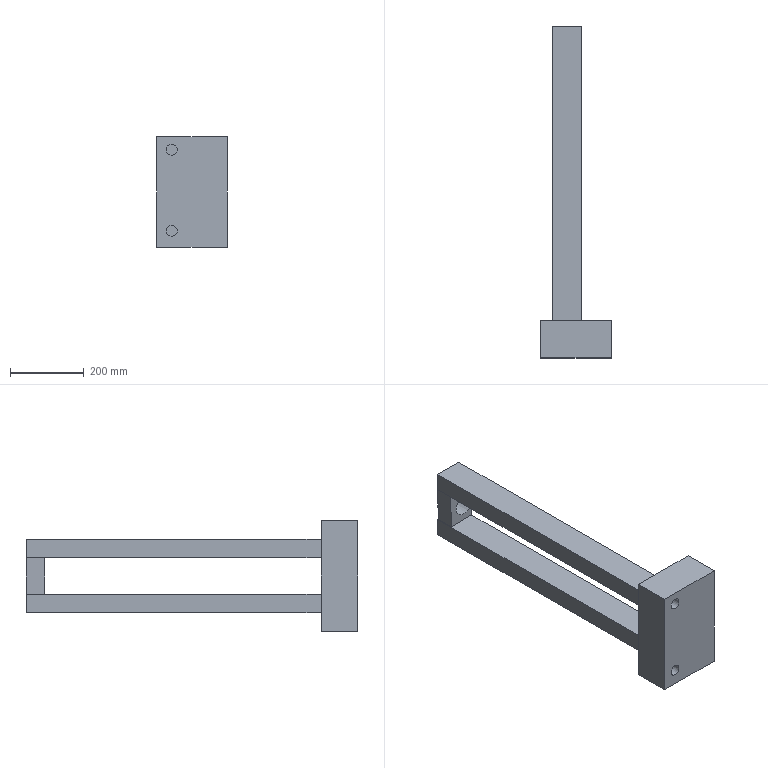Component | NX | UPPER_SUPPORT_SEAT_2 | 1 solid | 24 faces | volume 12324690 mm3 | plane 21 | cylinder 3 | commonest cylinder face diameters 30 x2 60 x1